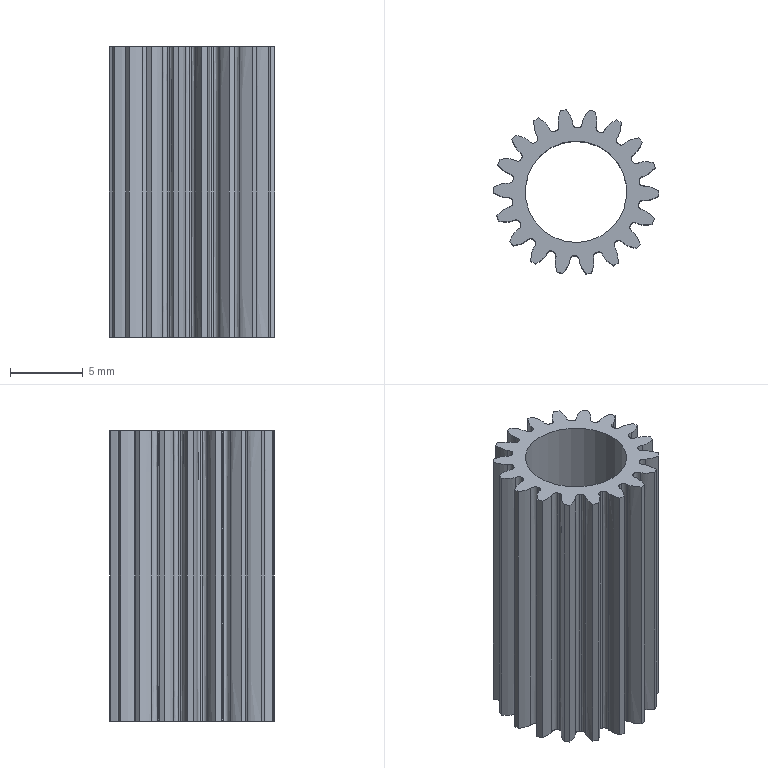Component | NX | GEAR | 1 solid | 111 faces | volume 851 mm3 | other 90 | cylinder 19 | plane 2 | commonest cylinder face diameters 8.835 x18 7 x1